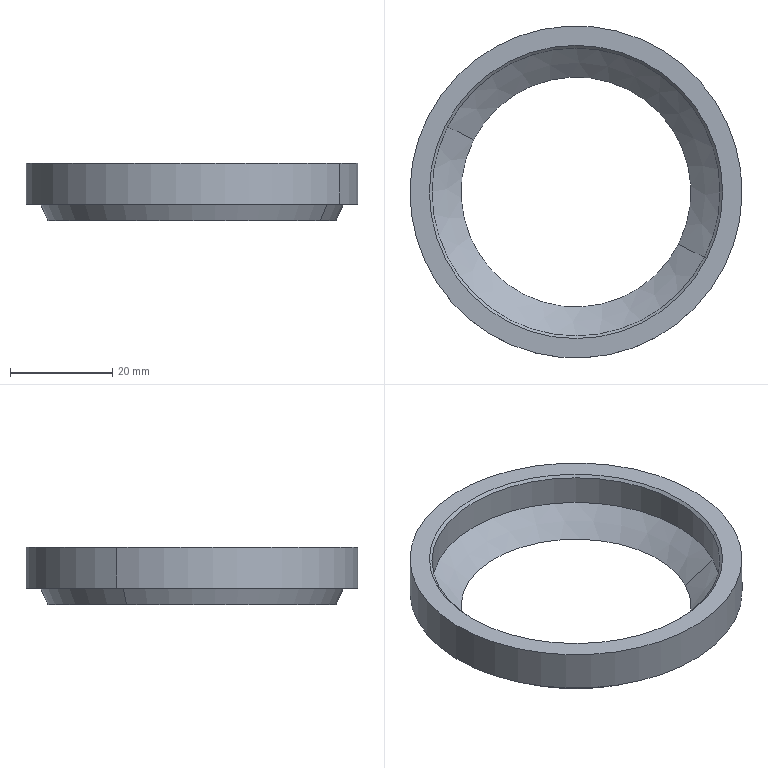Component | SolidWorks | GB_T10708.3-1989TypeBRubberDustSealFB45_65_8-1 | 1 solid | 13 faces | box 65 x 65 x 11.2 mm | volume 9211 mm3 | cone 6 | cylinder 4 | plane 3 | commonest cylinder face diameters 65 x2 56.4 x2
build123d program:
from build123d import *

# Parameters (mm, degrees)
CHAMFER1_SIZE = 0.5


with BuildPart() as part:
    # Sketch1 → Base-Revolve (revolve)
    with BuildSketch(Plane.XY, mode=Mode.PRIVATE) as base_revolve_sk:
        Polygon((22.5, 11.2), (28.2, 11.2), (29.633, 8), (32.5, 8), (32.5, 0), (28.2, 0), (28.2, 6.4), align=None)
    revolve(base_revolve_sk.sketch.rotate(Axis((0, 0, 0), (0, 1, 0)), 90), axis=Axis((0, 0, 0), (0, 1, 0)))

    # Chamfer1
    chamfer1_edges = [part.edges().sort_by_distance(p)[0] for p in [
        (0, 0, 28.2),
    ]]
    chamfer(chamfer1_edges, length=CHAMFER1_SIZE)


solid = part.part

# Placed as in the assembly
solid = solid.moved(Location((-30, 0, -104.5), (-90, 0, 0)))
STEP:
#1=COLOUR_RGB('',0.7922,0.8196,0.9333);
#2=FILL_AREA_STYLE_COLOUR('',#1);
#3=FILL_AREA_STYLE('',(#2));
#4=SURFACE_STYLE_FILL_AREA(#3);
#5=SURFACE_SIDE_STYLE('',(#4));
#6=SURFACE_STYLE_USAGE(.BOTH.,#5);
#7=PRESENTATION_STYLE_ASSIGNMENT((#6));
#8=CARTESIAN_POINT('',(-2.17,0.5043,-4.134));
#9=VERTEX_POINT('',#8);
#10=CARTESIAN_POINT('',(-0.192,-0.5043,-4.134));
#11=VERTEX_POINT('',#10);
#12=CARTESIAN_POINT('',(-1.181,0.,-4.134));
#13=DIRECTION('',(-0.,-0.,1.));
#14=DIRECTION('',(0.8909,-0.4543,0.));
#15=AXIS2_PLACEMENT_3D('',#12,#13,#14);
#16=CIRCLE('',#15,1.11);
#17=EDGE_CURVE('',#9,#11,#16,.T.);
#18=ORIENTED_EDGE('',*,*,#17,.F.);
#19=CARTESIAN_POINT('',(-2.188,0.5133,-4.114));
#20=VERTEX_POINT('',#19);
#21=CARTESIAN_POINT('',(-2.17,0.5043,-4.134));
#22=DIRECTION('',(-0.6299,0.3212,0.7071));
#23=VECTOR('',#22,39.37);
#24=LINE('',#21,#23);
#25=EDGE_CURVE('',#9,#20,#24,.T.);
#26=ORIENTED_EDGE('',*,*,#25,.T.);
#27=CARTESIAN_POINT('',(-0.1745,-0.5133,-4.114));
#28=VERTEX_POINT('',#27);
#29=CARTESIAN_POINT('',(-1.181,0.,-4.114));
#30=DIRECTION('',(0.,0.,-1.));
#31=DIRECTION('',(0.8909,-0.4543,0.));
#32=AXIS2_PLACEMENT_3D('',#29,#30,#31);
#33=CIRCLE('',#32,1.13);
#34=EDGE_CURVE('',#28,#20,#33,.T.);
#35=ORIENTED_EDGE('',*,*,#34,.F.);
#36=CARTESIAN_POINT('',(-0.192,-0.5043,-4.134));
#37=DIRECTION('',(0.6299,-0.3212,0.7071));
#38=VECTOR('',#37,39.37);
#39=LINE('',#36,#38);
#40=EDGE_CURVE('',#11,#28,#39,.T.);
#41=ORIENTED_EDGE('',*,*,#40,.F.);
#42=EDGE_LOOP('',(#18,#26,#35,#41));
#43=FACE_OUTER_BOUND('',#42,.T.);
#44=CARTESIAN_POINT('',(-1.181,0.,-4.134));
#45=DIRECTION('',(-0.,-0.,1.));
#46=DIRECTION('',(0.8909,-0.4543,0.));
#47=AXIS2_PLACEMENT_3D('',#44,#45,#46);
#48=CONICAL_SURFACE('',#47,1.11,0.7854);
#49=ADVANCED_FACE('',(#43),#48,.F.);
#50=CARTESIAN_POINT('',(-0.192,-0.5043,-4.555));
#51=VERTEX_POINT('',#50);
#52=CARTESIAN_POINT('',(-2.17,0.5043,-4.555));
#53=VERTEX_POINT('',#52);
#54=CARTESIAN_POINT('',(-1.181,0.,-4.555));
#55=DIRECTION('',(-0.,-0.,1.));
#56=DIRECTION('',(0.8909,-0.4543,0.));
#57=AXIS2_PLACEMENT_3D('',#54,#55,#56);
#58=CIRCLE('',#57,1.11);
#59=EDGE_CURVE('',#51,#53,#58,.T.);
#60=ORIENTED_EDGE('',*,*,#59,.T.);
#61=CARTESIAN_POINT('',(-2.22,0.53,-4.429));
#62=VERTEX_POINT('',#61);
#63=CARTESIAN_POINT('',(-2.22,0.53,-4.429));
#64=DIRECTION('',(-0.3642,0.1857,0.9126));
#65=VECTOR('',#64,39.37);
#66=LINE('',#63,#65);
#67=EDGE_CURVE('',#53,#62,#66,.T.);
#68=ORIENTED_EDGE('',*,*,#67,.T.);
#69=CARTESIAN_POINT('',(-0.1418,-0.53,-4.429));
#70=VERTEX_POINT('',#69);
#71=CARTESIAN_POINT('',(-1.181,0.,-4.429));
#72=DIRECTION('',(-0.,-0.,1.));
#73=DIRECTION('',(0.8909,-0.4543,0.));
#74=AXIS2_PLACEMENT_3D('',#71,#72,#73);
#75=CIRCLE('',#74,1.167);
#76=EDGE_CURVE('',#70,#62,#75,.T.);
#77=ORIENTED_EDGE('',*,*,#76,.F.);
#78=CARTESIAN_POINT('',(-0.1418,-0.53,-4.429));
#79=DIRECTION('',(0.3642,-0.1857,0.9126));
#80=VECTOR('',#79,39.37);
#81=LINE('',#78,#80);
#82=EDGE_CURVE('',#51,#70,#81,.T.);
#83=ORIENTED_EDGE('',*,*,#82,.F.);
#84=EDGE_LOOP('',(#60,#68,#77,#83));
#85=FACE_OUTER_BOUND('',#84,.T.);
#86=CARTESIAN_POINT('',(-1.181,0.,-4.429));
#87=DIRECTION('',(-0.,-0.,1.));
#88=DIRECTION('',(0.8909,-0.4543,0.));
#89=AXIS2_PLACEMENT_3D('',#86,#87,#88);
#90=CONICAL_SURFACE('',#89,1.167,0.4211);
#91=ADVANCED_FACE('',(#85),#90,.T.);
#92=CARTESIAN_POINT('',(-0.04121,-0.5812,-4.429));
#93=VERTEX_POINT('',#92);
#94=CARTESIAN_POINT('',(-2.321,0.5812,-4.429));
#95=VERTEX_POINT('',#94);
#96=CARTESIAN_POINT('',(-1.181,0.,-4.429));
#97=DIRECTION('',(-0.,-0.,1.));
#98=DIRECTION('',(0.8909,-0.4543,0.));
#99=AXIS2_PLACEMENT_3D('',#96,#97,#98);
#100=CIRCLE('',#99,1.28);
#101=EDGE_CURVE('',#93,#95,#100,.T.);
#102=ORIENTED_EDGE('',*,*,#101,.T.);
#103=CARTESIAN_POINT('',(-2.321,0.5812,-4.114));
#104=VERTEX_POINT('',#103);
#105=CARTESIAN_POINT('',(-2.321,0.5812,-4.114));
#106=DIRECTION('',(-0.,-0.,1.));
#107=VECTOR('',#106,39.37);
#108=LINE('',#105,#107);
#109=EDGE_CURVE('',#95,#104,#108,.T.);
#110=ORIENTED_EDGE('',*,*,#109,.T.);
#111=CARTESIAN_POINT('',(-0.04121,-0.5812,-4.114));
#112=VERTEX_POINT('',#111);
#113=CARTESIAN_POINT('',(-1.181,0.,-4.114));
#114=DIRECTION('',(-0.,-0.,1.));
#115=DIRECTION('',(0.8909,-0.4543,0.));
#116=AXIS2_PLACEMENT_3D('',#113,#114,#115);
#117=CIRCLE('',#116,1.28);
#118=EDGE_CURVE('',#112,#104,#117,.T.);
#119=ORIENTED_EDGE('',*,*,#118,.F.);
#120=CARTESIAN_POINT('',(-0.04121,-0.5812,-4.114));
#121=DIRECTION('',(-0.,-0.,1.));
#122=VECTOR('',#121,39.37);
#123=LINE('',#120,#122);
#124=EDGE_CURVE('',#93,#112,#123,.T.);
#125=ORIENTED_EDGE('',*,*,#124,.F.);
#126=EDGE_LOOP('',(#102,#110,#119,#125));
#127=FACE_OUTER_BOUND('',#126,.T.);
#128=CARTESIAN_POINT('',(-1.181,0.,-4.114));
#129=DIRECTION('',(-0.,-0.,1.));
#130=DIRECTION('',(0.8909,-0.4543,0.));
#131=AXIS2_PLACEMENT_3D('',#128,#129,#130);
#132=CYLINDRICAL_SURFACE('',#131,1.28);
#133=ADVANCED_FACE('',(#127),#132,.T.);
#134=CARTESIAN_POINT('',(-2.17,0.5043,-4.366));
#135=VERTEX_POINT('',#134);
#136=CARTESIAN_POINT('',(-0.192,-0.5043,-4.366));
#137=VERTEX_POINT('',#136);
#138=CARTESIAN_POINT('',(-1.181,0.,-4.366));
#139=DIRECTION('',(-0.,-0.,1.));
#140=DIRECTION('',(0.8909,-0.4543,0.));
#141=AXIS2_PLACEMENT_3D('',#138,#139,#140);
#142=CIRCLE('',#141,1.11);
#143=EDGE_CURVE('',#135,#137,#142,.T.);
#144=ORIENTED_EDGE('',*,*,#143,.F.);
#145=CARTESIAN_POINT('',(-2.17,0.5043,-4.114));
#146=DIRECTION('',(-0.,-0.,1.));
#147=VECTOR('',#146,39.37);
#148=LINE('',#145,#147);
#149=EDGE_CURVE('',#135,#9,#148,.T.);
#150=ORIENTED_EDGE('',*,*,#149,.T.);
#151=ORIENTED_EDGE('',*,*,#17,.T.);
#152=CARTESIAN_POINT('',(-0.192,-0.5043,-4.114));
#153=DIRECTION('',(-0.,-0.,1.));
#154=VECTOR('',#153,39.37);
#155=LINE('',#152,#154);
#156=EDGE_CURVE('',#137,#11,#155,.T.);
#157=ORIENTED_EDGE('',*,*,#156,.F.);
#158=EDGE_LOOP('',(#144,#150,#151,#157));
#159=FACE_OUTER_BOUND('',#158,.T.);
#160=CARTESIAN_POINT('',(-1.181,0.,-4.114));
#161=DIRECTION('',(-0.,-0.,1.));
#162=DIRECTION('',(0.8909,-0.4543,0.));
#163=AXIS2_PLACEMENT_3D('',#160,#161,#162);
#164=CYLINDRICAL_SURFACE('',#163,1.11);
#165=ADVANCED_FACE('',(#159),#164,.F.);
#166=CARTESIAN_POINT('',(-1.97,0.4024,-4.555));
#167=VERTEX_POINT('',#166);
#168=CARTESIAN_POINT('',(-0.3919,-0.4024,-4.555));
#169=VERTEX_POINT('',#168);
#170=CARTESIAN_POINT('',(-1.181,0.,-4.555));
#171=DIRECTION('',(-0.,-0.,1.));
#172=DIRECTION('',(0.8909,-0.4543,0.));
#173=AXIS2_PLACEMENT_3D('',#170,#171,#172);
#174=CIRCLE('',#173,0.8858);
#175=EDGE_CURVE('',#167,#169,#174,.T.);
#176=ORIENTED_EDGE('',*,*,#175,.F.);
#177=CARTESIAN_POINT('',(-1.97,0.4024,-4.555));
#178=DIRECTION('',(-0.6814,0.3475,0.6441));
#179=VECTOR('',#178,39.37);
#180=LINE('',#177,#179);
#181=EDGE_CURVE('',#167,#135,#180,.T.);
#182=ORIENTED_EDGE('',*,*,#181,.T.);
#183=ORIENTED_EDGE('',*,*,#143,.T.);
#184=CARTESIAN_POINT('',(-0.3919,-0.4024,-4.555));
#185=DIRECTION('',(0.6814,-0.3475,0.6441));
#186=VECTOR('',#185,39.37);
#187=LINE('',#184,#186);
#188=EDGE_CURVE('',#169,#137,#187,.T.);
#189=ORIENTED_EDGE('',*,*,#188,.F.);
#190=EDGE_LOOP('',(#176,#182,#183,#189));
#191=FACE_OUTER_BOUND('',#190,.T.);
#192=CARTESIAN_POINT('',(-1.181,0.,-4.555));
#193=DIRECTION('',(-0.,-0.,1.));
#194=DIRECTION('',(0.8909,-0.4543,0.));
#195=AXIS2_PLACEMENT_3D('',#192,#193,#194);
#196=CONICAL_SURFACE('',#195,0.8858,0.8709);
#197=ADVANCED_FACE('',(#191),#196,.F.);
#198=ORIENTED_EDGE('',*,*,#181,.F.);
#199=CARTESIAN_POINT('',(-1.181,0.,-4.555));
#200=DIRECTION('',(-0.,-0.,1.));
#201=DIRECTION('',(0.8909,-0.4543,0.));
#202=AXIS2_PLACEMENT_3D('',#199,#200,#201);
#203=CIRCLE('',#202,0.8858);
#204=EDGE_CURVE('',#169,#167,#203,.T.);
#205=ORIENTED_EDGE('',*,*,#204,.F.);
#206=ORIENTED_EDGE('',*,*,#188,.T.);
#207=CARTESIAN_POINT('',(-1.181,0.,-4.366));
#208=DIRECTION('',(-0.,-0.,1.));
#209=DIRECTION('',(0.8909,-0.4543,0.));
#210=AXIS2_PLACEMENT_3D('',#207,#208,#209);
#211=CIRCLE('',#210,1.11);
#212=EDGE_CURVE('',#137,#135,#211,.T.);
#213=ORIENTED_EDGE('',*,*,#212,.T.);
#214=EDGE_LOOP('',(#198,#205,#206,#213));
#215=FACE_OUTER_BOUND('',#214,.T.);
#216=CARTESIAN_POINT('',(-1.181,0.,-4.555));
#217=DIRECTION('',(-0.,-0.,1.));
#218=DIRECTION('',(0.8909,-0.4543,0.));
#219=AXIS2_PLACEMENT_3D('',#216,#217,#218);
#220=CONICAL_SURFACE('',#219,0.8858,0.8709);
#221=ADVANCED_FACE('',(#215),#220,.F.);
#222=ORIENTED_EDGE('',*,*,#149,.F.);
#223=ORIENTED_EDGE('',*,*,#212,.F.);
#224=ORIENTED_EDGE('',*,*,#156,.T.);
#225=CARTESIAN_POINT('',(-1.181,0.,-4.134));
#226=DIRECTION('',(-0.,-0.,1.));
#227=DIRECTION('',(0.8909,-0.4543,0.));
#228=AXIS2_PLACEMENT_3D('',#225,#226,#227);
#229=CIRCLE('',#228,1.11);
#230=EDGE_CURVE('',#11,#9,#229,.T.);
#231=ORIENTED_EDGE('',*,*,#230,.T.);
#232=EDGE_LOOP('',(#222,#223,#224,#231));
#233=FACE_OUTER_BOUND('',#232,.T.);
#234=CARTESIAN_POINT('',(-1.181,0.,-4.114));
#235=DIRECTION('',(-0.,-0.,1.));
#236=DIRECTION('',(0.8909,-0.4543,0.));
#237=AXIS2_PLACEMENT_3D('',#234,#235,#236);
#238=CYLINDRICAL_SURFACE('',#237,1.11);
#239=ADVANCED_FACE('',(#233),#238,.F.);
#240=ORIENTED_EDGE('',*,*,#34,.T.);
#241=CARTESIAN_POINT('',(-1.181,0.,-4.114));
#242=DIRECTION('',(0.,0.,-1.));
#243=DIRECTION('',(0.8909,-0.4543,0.));
#244=AXIS2_PLACEMENT_3D('',#241,#242,#243);
#245=CIRCLE('',#244,1.13);
#246=EDGE_CURVE('',#20,#28,#245,.T.);
#247=ORIENTED_EDGE('',*,*,#246,.T.);
#248=EDGE_LOOP('',(#240,#247));
#249=FACE_BOUND('',#248,.T.);
#250=ORIENTED_EDGE('',*,*,#118,.T.);
#251=CARTESIAN_POINT('',(-1.181,0.,-4.114));
#252=DIRECTION('',(-0.,-0.,1.));
#253=DIRECTION('',(0.8909,-0.4543,0.));
#254=AXIS2_PLACEMENT_3D('',#251,#252,#253);
#255=CIRCLE('',#254,1.28);
#256=EDGE_CURVE('',#104,#112,#255,.T.);
#257=ORIENTED_EDGE('',*,*,#256,.T.);
#258=EDGE_LOOP('',(#250,#257));
#259=FACE_OUTER_BOUND('',#258,.T.);
#260=CARTESIAN_POINT('',(-0.5999,1.14,-4.114));
#261=DIRECTION('',(-0.,-0.,1.));
#262=DIRECTION('',(0.8909,-0.4543,0.));
#263=AXIS2_PLACEMENT_3D('',#260,#261,#262);
#264=PLANE('',#263);
#265=ADVANCED_FACE('',(#249,#259),#264,.T.);
#266=ORIENTED_EDGE('',*,*,#109,.F.);
#267=CARTESIAN_POINT('',(-1.181,0.,-4.429));
#268=DIRECTION('',(-0.,-0.,1.));
#269=DIRECTION('',(0.8909,-0.4543,0.));
#270=AXIS2_PLACEMENT_3D('',#267,#268,#269);
#271=CIRCLE('',#270,1.28);
#272=EDGE_CURVE('',#95,#93,#271,.T.);
#273=ORIENTED_EDGE('',*,*,#272,.T.);
#274=ORIENTED_EDGE('',*,*,#124,.T.);
#275=ORIENTED_EDGE('',*,*,#256,.F.);
#276=EDGE_LOOP('',(#266,#273,#274,#275));
#277=FACE_OUTER_BOUND('',#276,.T.);
#278=CARTESIAN_POINT('',(-1.181,0.,-4.114));
#279=DIRECTION('',(-0.,-0.,1.));
#280=DIRECTION('',(0.8909,-0.4543,0.));
#281=AXIS2_PLACEMENT_3D('',#278,#279,#280);
#282=CYLINDRICAL_SURFACE('',#281,1.28);
#283=ADVANCED_FACE('',(#277),#282,.T.);
#284=ORIENTED_EDGE('',*,*,#76,.T.);
#285=CARTESIAN_POINT('',(-1.181,0.,-4.429));
#286=DIRECTION('',(-0.,-0.,1.));
#287=DIRECTION('',(0.8909,-0.4543,0.));
#288=AXIS2_PLACEMENT_3D('',#285,#286,#287);
#289=CIRCLE('',#288,1.167);
#290=EDGE_CURVE('',#62,#70,#289,.T.);
#291=ORIENTED_EDGE('',*,*,#290,.T.);
#292=EDGE_LOOP('',(#284,#291));
#293=FACE_BOUND('',#292,.T.);
#294=ORIENTED_EDGE('',*,*,#101,.F.);
#295=ORIENTED_EDGE('',*,*,#272,.F.);
#296=EDGE_LOOP('',(#294,#295));
#297=FACE_OUTER_BOUND('',#296,.T.);
#298=CARTESIAN_POINT('',(-0.6511,1.039,-4.429));
#299=DIRECTION('',(0.,0.,-1.));
#300=DIRECTION('',(-0.8909,0.4543,-0.));
#301=AXIS2_PLACEMENT_3D('',#298,#299,#300);
#302=PLANE('',#301);
#303=ADVANCED_FACE('',(#293,#297),#302,.T.);
#304=ORIENTED_EDGE('',*,*,#67,.F.);
#305=CARTESIAN_POINT('',(-1.181,0.,-4.555));
#306=DIRECTION('',(-0.,-0.,1.));
#307=DIRECTION('',(0.8909,-0.4543,0.));
#308=AXIS2_PLACEMENT_3D('',#305,#306,#307);
#309=CIRCLE('',#308,1.11);
#310=EDGE_CURVE('',#53,#51,#309,.T.);
#311=ORIENTED_EDGE('',*,*,#310,.T.);
#312=ORIENTED_EDGE('',*,*,#82,.T.);
#313=ORIENTED_EDGE('',*,*,#290,.F.);
#314=EDGE_LOOP('',(#304,#311,#312,#313));
#315=FACE_OUTER_BOUND('',#314,.T.);
#316=CARTESIAN_POINT('',(-1.181,0.,-4.429));
#317=DIRECTION('',(-0.,-0.,1.));
#318=DIRECTION('',(0.8909,-0.4543,0.));
#319=AXIS2_PLACEMENT_3D('',#316,#317,#318);
#320=CONICAL_SURFACE('',#319,1.167,0.4211);
#321=ADVANCED_FACE('',(#315),#320,.T.);
#322=ORIENTED_EDGE('',*,*,#204,.T.);
#323=ORIENTED_EDGE('',*,*,#175,.T.);
#324=EDGE_LOOP('',(#322,#323));
#325=FACE_BOUND('',#324,.T.);
#326=ORIENTED_EDGE('',*,*,#59,.F.);
#327=ORIENTED_EDGE('',*,*,#310,.F.);
#328=EDGE_LOOP('',(#326,#327));
#329=FACE_OUTER_BOUND('',#328,.T.);
#330=CARTESIAN_POINT('',(-0.7787,0.7892,-4.555));
#331=DIRECTION('',(0.,0.,-1.));
#332=DIRECTION('',(-0.8909,0.4543,-0.));
#333=AXIS2_PLACEMENT_3D('',#330,#331,#332);
#334=PLANE('',#333);
#335=ADVANCED_FACE('',(#325,#329),#334,.T.);
#336=ORIENTED_EDGE('',*,*,#25,.F.);
#337=ORIENTED_EDGE('',*,*,#230,.F.);
#338=ORIENTED_EDGE('',*,*,#40,.T.);
#339=ORIENTED_EDGE('',*,*,#246,.F.);
#340=EDGE_LOOP('',(#336,#337,#338,#339));
#341=FACE_OUTER_BOUND('',#340,.T.);
#342=CARTESIAN_POINT('',(-1.181,0.,-4.134));
#343=DIRECTION('',(-0.,-0.,1.));
#344=DIRECTION('',(0.8909,-0.4543,0.));
#345=AXIS2_PLACEMENT_3D('',#342,#343,#344);
#346=CONICAL_SURFACE('',#345,1.11,0.7854);
#347=ADVANCED_FACE('',(#341),#346,.F.);
#348=CLOSED_SHELL('',(#49,#91,#133,#165,#197,#221,#239,#265,#283,#303,#321,#335,#347));
#349=MANIFOLD_SOLID_BREP('',#348);
#350=STYLED_ITEM('',(#7),#349);
#351=(LENGTH_UNIT()NAMED_UNIT(*)SI_UNIT($,.METRE.));
#352=LENGTH_MEASURE_WITH_UNIT(LENGTH_MEASURE(0.0254),#351);
#353=DIMENSIONAL_EXPONENTS(1.,0.,0.,0.,0.,0.,0.);
#354=(CONVERSION_BASED_UNIT('',#352)LENGTH_UNIT()NAMED_UNIT(#353));
#355=UNCERTAINTY_MEASURE_WITH_UNIT(LENGTH_MEASURE(0.00001),#354,'','');
#356=(NAMED_UNIT(*)PLANE_ANGLE_UNIT()SI_UNIT($,.RADIAN.));
#357=(NAMED_UNIT(*)SI_UNIT($,.STERADIAN.)SOLID_ANGLE_UNIT());
#358=(GEOMETRIC_REPRESENTATION_CONTEXT(3)GLOBAL_UNCERTAINTY_ASSIGNED_CONTEXT((#355))GLOBAL_UNIT_ASSIGNED_CONTEXT((#354,#356,#357))REPRESENTATION_CONTEXT('',''));
#359=MECHANICAL_DESIGN_GEOMETRIC_PRESENTATION_REPRESENTATION('',(#350),#358);
#360=CARTESIAN_POINT('',(0.,0.,0.));
#361=DIRECTION('',(0.,0.,1.));
#362=DIRECTION('',(1.,0.,0.));
#363=AXIS2_PLACEMENT_3D('',#360,#361,#362);
#364=(LENGTH_UNIT()NAMED_UNIT(*)SI_UNIT($,.METRE.));
#365=LENGTH_MEASURE_WITH_UNIT(LENGTH_MEASURE(0.0254),#364);
#366=DIMENSIONAL_EXPONENTS(1.,0.,0.,0.,0.,0.,0.);
#367=(CONVERSION_BASED_UNIT('',#365)LENGTH_UNIT()NAMED_UNIT(#366));
#368=UNCERTAINTY_MEASURE_WITH_UNIT(LENGTH_MEASURE(0.00001),#367,'','');
#369=(NAMED_UNIT(*)PLANE_ANGLE_UNIT()SI_UNIT($,.RADIAN.));
#370=(NAMED_UNIT(*)SI_UNIT($,.STERADIAN.)SOLID_ANGLE_UNIT());
#371=(GEOMETRIC_REPRESENTATION_CONTEXT(3)GLOBAL_UNCERTAINTY_ASSIGNED_CONTEXT((#368))GLOBAL_UNIT_ASSIGNED_CONTEXT((#367,#369,#370))REPRESENTATION_CONTEXT('',''));
#372=ADVANCED_BREP_SHAPE_REPRESENTATION('',(#349,#363),#371);
#373=PRESENTATION_LAYER_ASSIGNMENT('','',(#350));